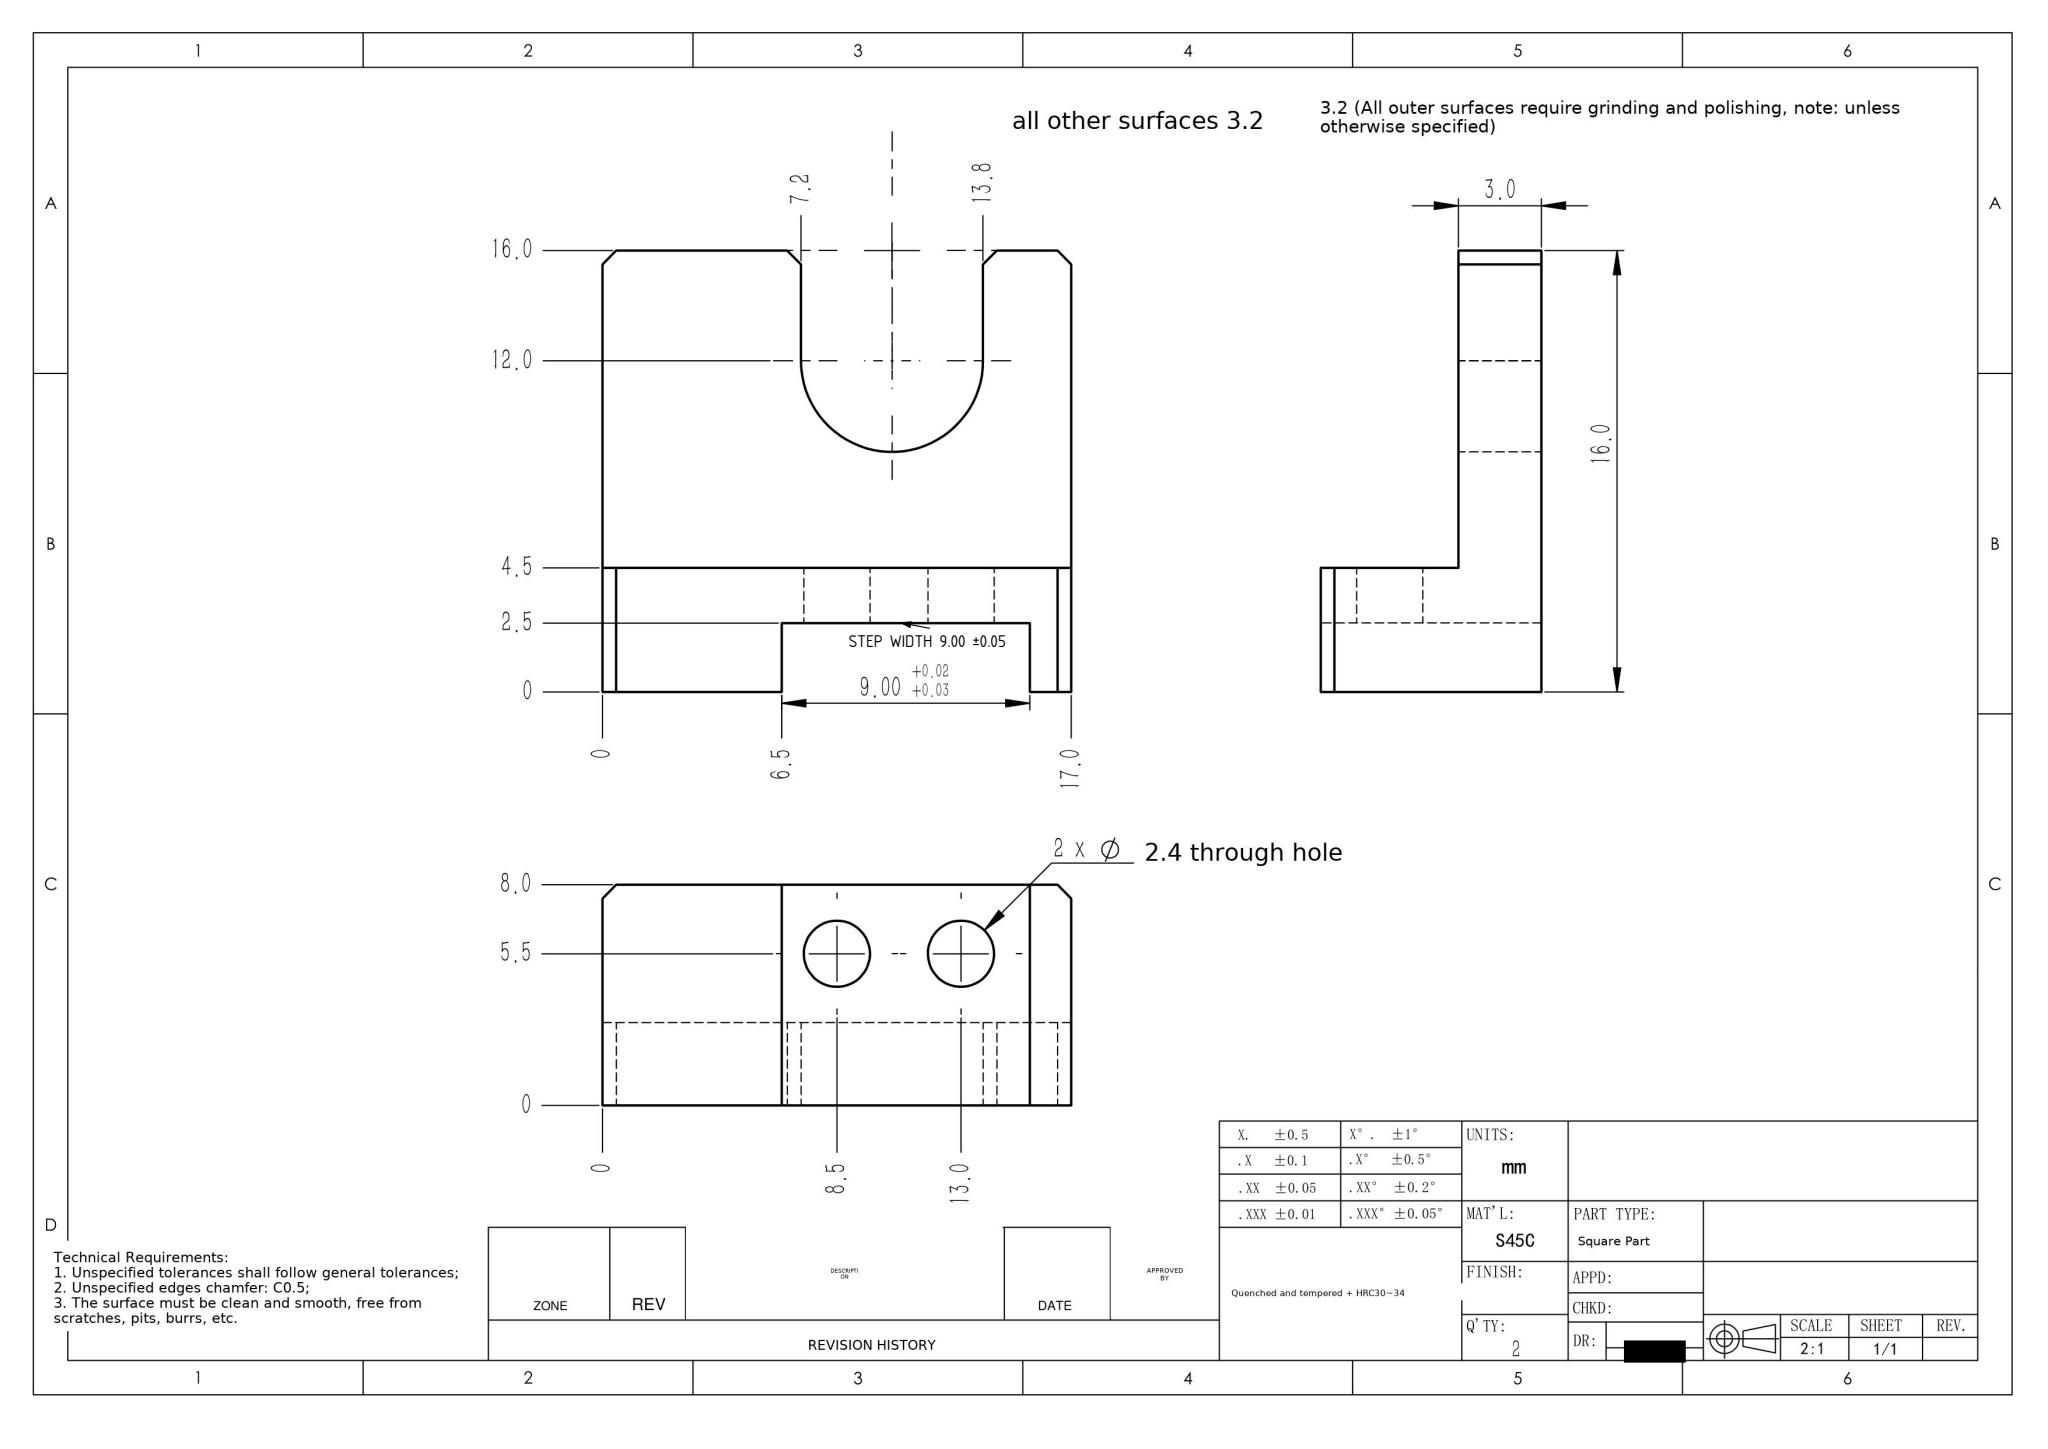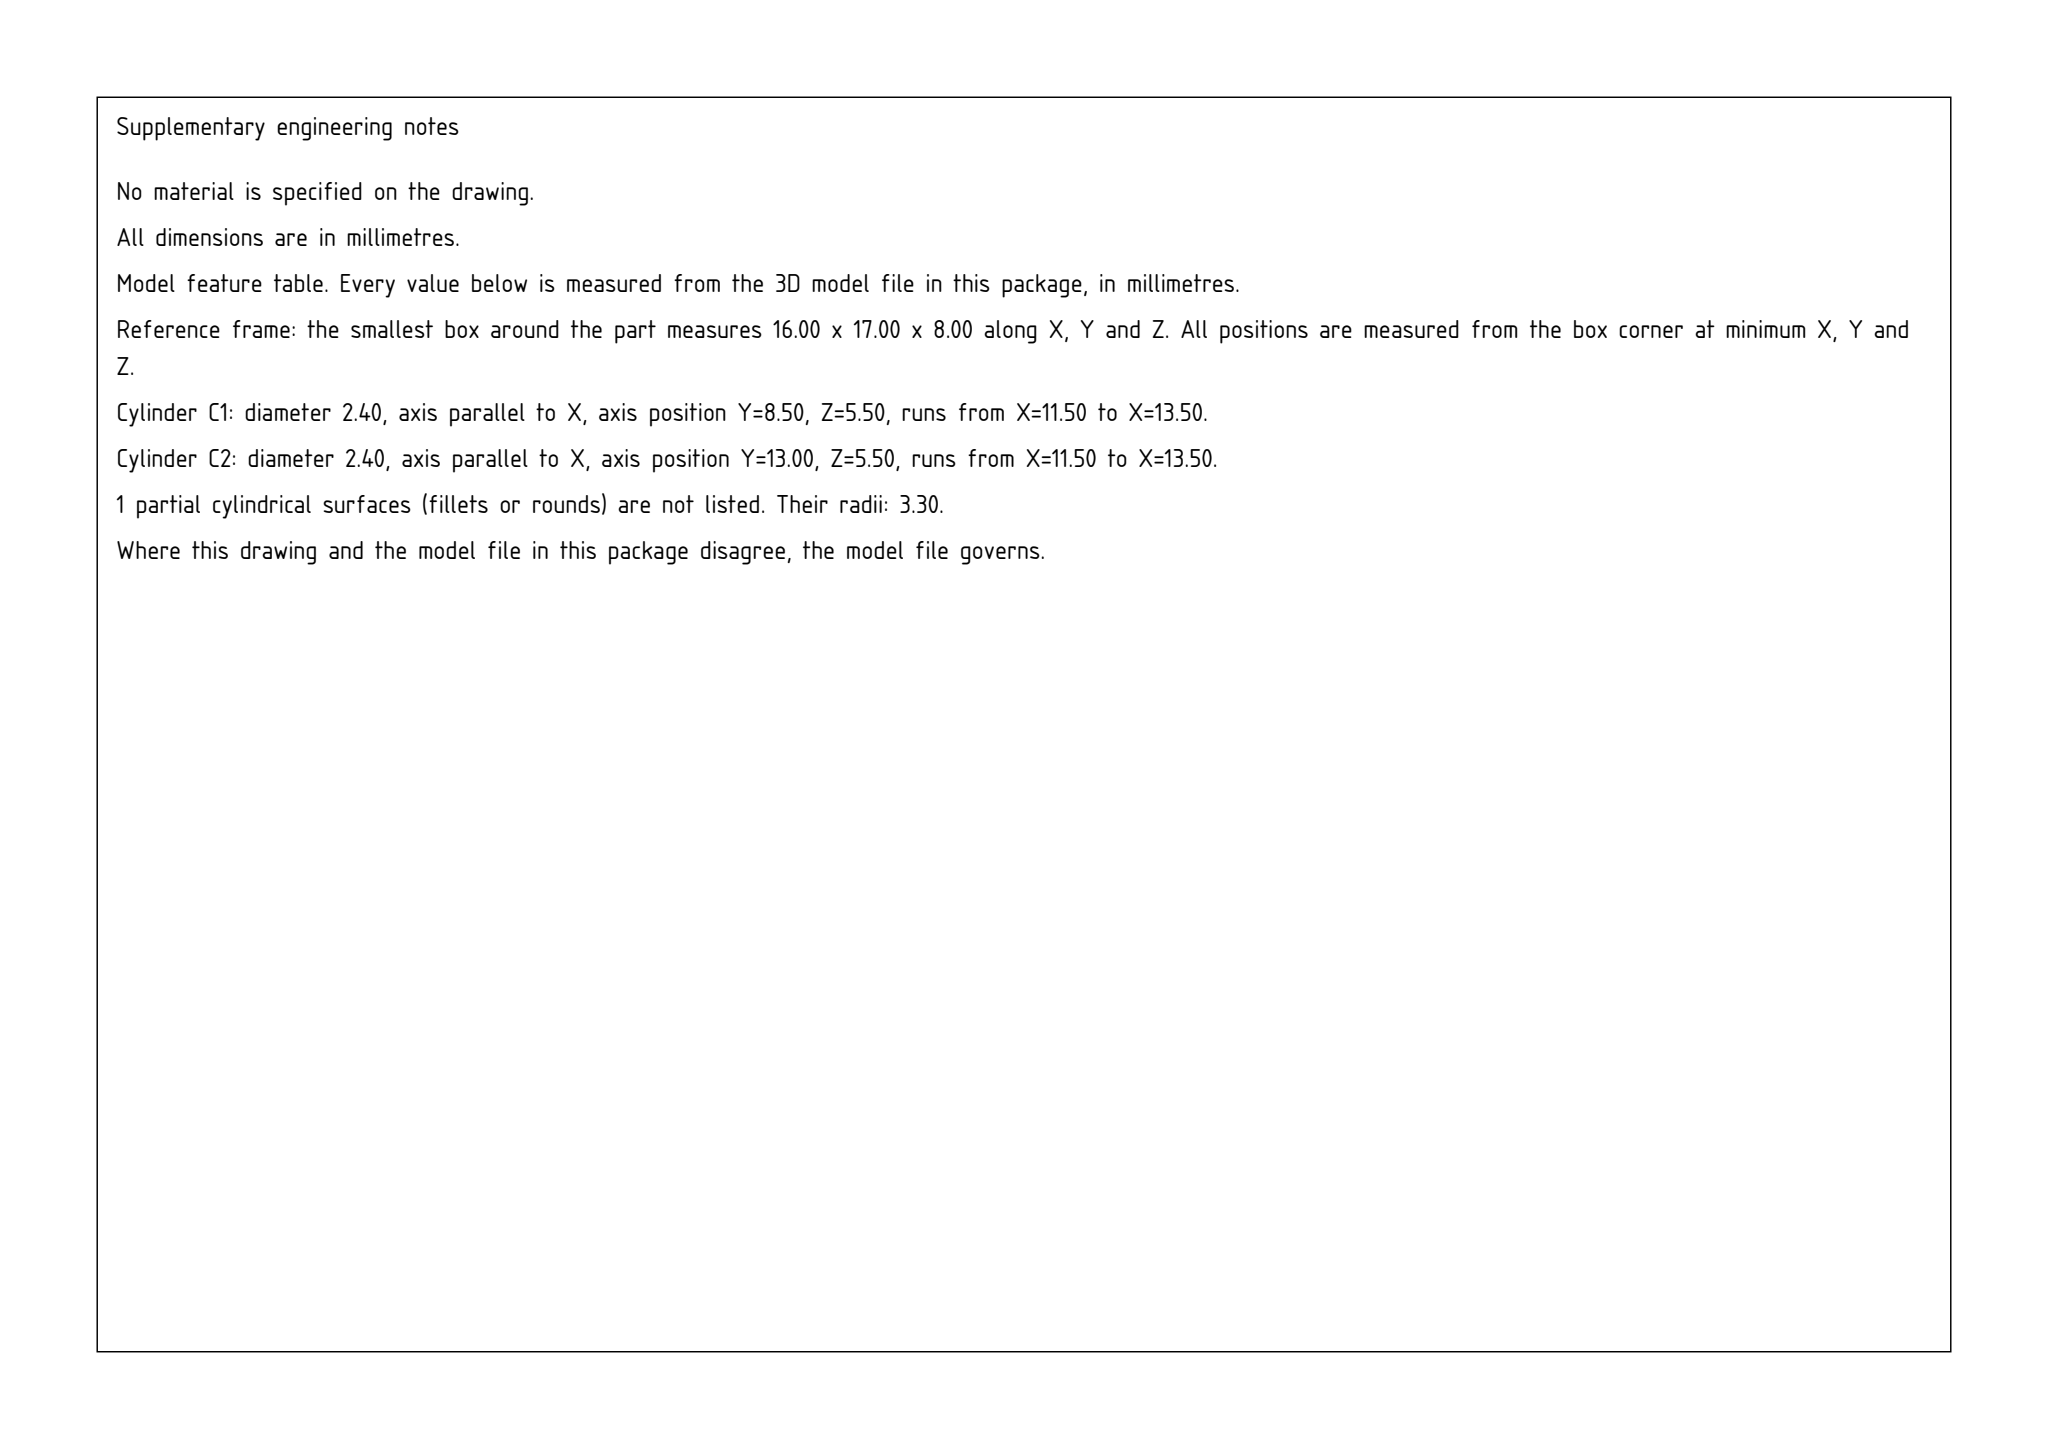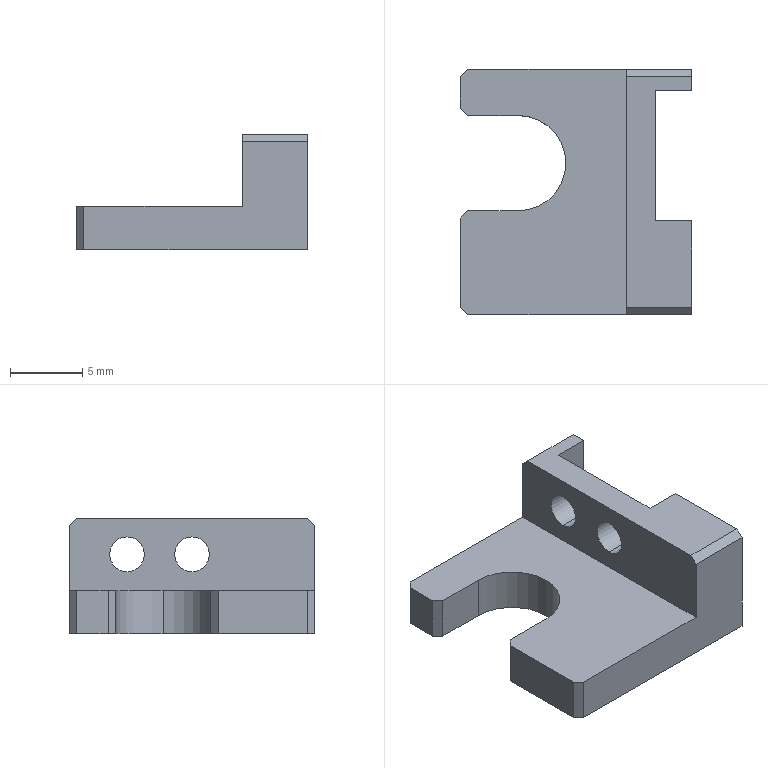Part | SolidWorks | mm | material S45C | 1 solid | 27 faces | box 16 x 17 x 8 mm | volume 867 mm3 | plane 21 | cylinder 6 | commonest cylinder face diameters 2.4 x4 6.6 x2
Drawing notes:
FRONT VIEW: STEP WIDTH 9.00 (FROM 6.5 TO 15.5), TOL ±0.05 | from the solid: Planes y=6.5 and y=15.5 (x 13.5-16.0, z 0-8) give step width 15.5-6.5=9.00; .XX tol block ±0.05
build123d program:
from build123d import *

# Parameters (mm, degrees)
SKETCH1_W            = 16
SKETCH1_H            = 17
BOSS_EXTRUDE1_DEPTH  = 8
SKETCH2_W            = 11.5
SKETCH2_H            = 17
CUT_EXTRUDE1_DEPTH   = 5
CUT_EXTRUDE2_DEPTH   = 19.795
SKETCH5_W            = 8
SKETCH5_H            = 9
CUT_EXTRUDE3_DEPTH   = 2.5
M2_CLEARANCE_HOLE1_D = 2.4
CHAMFER1_SIZE        = 0.5


with BuildPart() as part:
    # Sketch1 → Boss-Extrude1 (new body)
    with BuildSketch(Plane.XY):
        with Locations((-8, 0)):
            Rectangle(SKETCH1_W, SKETCH1_H)
    extrude(amount=BOSS_EXTRUDE1_DEPTH)

    # Sketch2 → Cut-Extrude1 (cut)
    with BuildSketch(Plane.XY.offset(8)):
        with Locations((-10.25, 0)):
            Rectangle(SKETCH2_W, SKETCH2_H)
    extrude(amount=-CUT_EXTRUDE1_DEPTH, mode=Mode.SUBTRACT)

    # Sketch3 → Cut-Extrude2 (cut, through all)
    with BuildSketch(Plane.XY.offset(3)):
        with BuildLine():
            Line((-16, 5.3), (-12, 5.3))
            ThreePointArc((-12, 5.3), (-8.7, 2), (-12, -1.3))
            Line((-12, -1.3), (-16, -1.3))
            ThreePointArc((-16, -1.3), (-19.3, 2), (-16, 5.3))
        make_face()
    extrude(amount=-CUT_EXTRUDE2_DEPTH, mode=Mode.SUBTRACT)

    # Sketch5 → Cut-Extrude3 (cut)
    with BuildSketch(Plane(origin=(0, 0, 0), x_dir=(0, 0, -1), z_dir=(1, 0, 0))):
        with Locations((-4, 2.5)):
            Rectangle(SKETCH5_W, SKETCH5_H)
    extrude(amount=-CUT_EXTRUDE3_DEPTH, mode=Mode.SUBTRACT)

    # M2 Clearance Hole1 (through all)
    with Locations(Plane.ZY.offset(4.5)):
        with Locations((5.5, 4.5), (5.5, 0)):
            Hole(M2_CLEARANCE_HOLE1_D / 2)

    # Chamfer1
    chamfer1_edges = [part.edges().sort_by_distance(p)[0] for p in [
        (-2.25, -8.5, 8),
        (-16, -8.5, 1.5),
        (-16, 8.5, 1.5),
        (-16, -1.3, 1.5),
        (-16, 5.3, 1.5),
        (-2.25, 8.5, 8),
    ]]
    chamfer(chamfer1_edges, length=CHAMFER1_SIZE)


solid = part.part
STEP:
#1=CARTESIAN_POINT('',(-2.5,4.5,4.3));
#2=VERTEX_POINT('',#1);
#3=CARTESIAN_POINT('',(-2.5,4.5,6.7));
#4=VERTEX_POINT('',#3);
#5=CARTESIAN_POINT('',(-2.5,4.5,5.5));
#6=DIRECTION('',(-1.,0.,0.));
#7=DIRECTION('',(0.,0.,1.));
#8=AXIS2_PLACEMENT_3D('',#5,#6,#7);
#9=CIRCLE('',#8,1.2);
#10=EDGE_CURVE('',#2,#4,#9,.T.);
#11=ORIENTED_EDGE('',*,*,#10,.F.);
#12=CARTESIAN_POINT('',(-4.5,4.5,4.3));
#13=VERTEX_POINT('',#12);
#14=CARTESIAN_POINT('',(-4.5,4.5,4.3));
#15=DIRECTION('',(-1.,0.,0.));
#16=VECTOR('',#15,1000.);
#17=LINE('',#14,#16);
#18=EDGE_CURVE('',#2,#13,#17,.T.);
#19=ORIENTED_EDGE('',*,*,#18,.T.);
#20=CARTESIAN_POINT('',(-4.5,4.5,6.7));
#21=VERTEX_POINT('',#20);
#22=CARTESIAN_POINT('',(-4.5,4.5,5.5));
#23=DIRECTION('',(-1.,0.,0.));
#24=DIRECTION('',(0.,0.,1.));
#25=AXIS2_PLACEMENT_3D('',#22,#23,#24);
#26=CIRCLE('',#25,1.2);
#27=EDGE_CURVE('',#13,#21,#26,.T.);
#28=ORIENTED_EDGE('',*,*,#27,.T.);
#29=CARTESIAN_POINT('',(-4.5,4.5,6.7));
#30=DIRECTION('',(-1.,0.,0.));
#31=VECTOR('',#30,1000.);
#32=LINE('',#29,#31);
#33=EDGE_CURVE('',#4,#21,#32,.T.);
#34=ORIENTED_EDGE('',*,*,#33,.F.);
#35=EDGE_LOOP('',(#11,#19,#28,#34));
#36=FACE_OUTER_BOUND('',#35,.T.);
#37=CARTESIAN_POINT('',(-4.5,4.5,5.5));
#38=DIRECTION('',(-1.,0.,0.));
#39=DIRECTION('',(0.,0.,1.));
#40=AXIS2_PLACEMENT_3D('',#37,#38,#39);
#41=CYLINDRICAL_SURFACE('',#40,1.2);
#42=ADVANCED_FACE('',(#36),#41,.F.);
#43=CARTESIAN_POINT('',(-2.5,0.,4.3));
#44=VERTEX_POINT('',#43);
#45=CARTESIAN_POINT('',(-2.5,0.,6.7));
#46=VERTEX_POINT('',#45);
#47=CARTESIAN_POINT('',(-2.5,0.,5.5));
#48=DIRECTION('',(-1.,0.,0.));
#49=DIRECTION('',(0.,0.,1.));
#50=AXIS2_PLACEMENT_3D('',#47,#48,#49);
#51=CIRCLE('',#50,1.2);
#52=EDGE_CURVE('',#44,#46,#51,.T.);
#53=ORIENTED_EDGE('',*,*,#52,.F.);
#54=CARTESIAN_POINT('',(-4.5,0.,4.3));
#55=VERTEX_POINT('',#54);
#56=CARTESIAN_POINT('',(-4.5,0.,4.3));
#57=DIRECTION('',(-1.,0.,0.));
#58=VECTOR('',#57,1000.);
#59=LINE('',#56,#58);
#60=EDGE_CURVE('',#44,#55,#59,.T.);
#61=ORIENTED_EDGE('',*,*,#60,.T.);
#62=CARTESIAN_POINT('',(-4.5,0.,6.7));
#63=VERTEX_POINT('',#62);
#64=CARTESIAN_POINT('',(-4.5,0.,5.5));
#65=DIRECTION('',(-1.,0.,0.));
#66=DIRECTION('',(0.,0.,1.));
#67=AXIS2_PLACEMENT_3D('',#64,#65,#66);
#68=CIRCLE('',#67,1.2);
#69=EDGE_CURVE('',#55,#63,#68,.T.);
#70=ORIENTED_EDGE('',*,*,#69,.T.);
#71=CARTESIAN_POINT('',(-4.5,0.,6.7));
#72=DIRECTION('',(-1.,0.,0.));
#73=VECTOR('',#72,1000.);
#74=LINE('',#71,#73);
#75=EDGE_CURVE('',#46,#63,#74,.T.);
#76=ORIENTED_EDGE('',*,*,#75,.F.);
#77=EDGE_LOOP('',(#53,#61,#70,#76));
#78=FACE_OUTER_BOUND('',#77,.T.);
#79=CARTESIAN_POINT('',(-4.5,0.,5.5));
#80=DIRECTION('',(-1.,0.,0.));
#81=DIRECTION('',(0.,0.,1.));
#82=AXIS2_PLACEMENT_3D('',#79,#80,#81);
#83=CYLINDRICAL_SURFACE('',#82,1.2);
#84=ADVANCED_FACE('',(#78),#83,.F.);
#85=CARTESIAN_POINT('',(-8.7,2.,0.));
#86=VERTEX_POINT('',#85);
#87=CARTESIAN_POINT('',(-12.,5.3,0.));
#88=VERTEX_POINT('',#87);
#89=CARTESIAN_POINT('',(-12.,2.,0.));
#90=DIRECTION('',(0.,0.,1.));
#91=DIRECTION('',(1.,0.,0.));
#92=AXIS2_PLACEMENT_3D('',#89,#90,#91);
#93=CIRCLE('',#92,3.3);
#94=EDGE_CURVE('',#86,#88,#93,.T.);
#95=ORIENTED_EDGE('',*,*,#94,.F.);
#96=CARTESIAN_POINT('',(-8.7,2.,3.));
#97=VERTEX_POINT('',#96);
#98=CARTESIAN_POINT('',(-8.7,2.,0.));
#99=DIRECTION('',(0.,0.,1.));
#100=VECTOR('',#99,1000.);
#101=LINE('',#98,#100);
#102=EDGE_CURVE('',#86,#97,#101,.T.);
#103=ORIENTED_EDGE('',*,*,#102,.T.);
#104=CARTESIAN_POINT('',(-12.,5.3,3.));
#105=VERTEX_POINT('',#104);
#106=CARTESIAN_POINT('',(-12.,2.,3.));
#107=DIRECTION('',(0.,0.,1.));
#108=DIRECTION('',(1.,0.,0.));
#109=AXIS2_PLACEMENT_3D('',#106,#107,#108);
#110=CIRCLE('',#109,3.3);
#111=EDGE_CURVE('',#97,#105,#110,.T.);
#112=ORIENTED_EDGE('',*,*,#111,.T.);
#113=CARTESIAN_POINT('',(-12.,5.3,0.));
#114=DIRECTION('',(0.,0.,1.));
#115=VECTOR('',#114,1000.);
#116=LINE('',#113,#115);
#117=EDGE_CURVE('',#88,#105,#116,.T.);
#118=ORIENTED_EDGE('',*,*,#117,.F.);
#119=EDGE_LOOP('',(#95,#103,#112,#118));
#120=FACE_OUTER_BOUND('',#119,.T.);
#121=CARTESIAN_POINT('',(-12.,2.,0.));
#122=DIRECTION('',(0.,0.,1.));
#123=DIRECTION('',(1.,0.,0.));
#124=AXIS2_PLACEMENT_3D('',#121,#122,#123);
#125=CYLINDRICAL_SURFACE('',#124,3.3);
#126=ADVANCED_FACE('',(#120),#125,.F.);
#127=CARTESIAN_POINT('',(0.,-8.,8.));
#128=VERTEX_POINT('',#127);
#129=CARTESIAN_POINT('',(0.,-2.,8.));
#130=VERTEX_POINT('',#129);
#131=CARTESIAN_POINT('',(0.,8.5,8.));
#132=DIRECTION('',(0.,1.,0.));
#133=VECTOR('',#132,1000.);
#134=LINE('',#131,#133);
#135=EDGE_CURVE('',#128,#130,#134,.T.);
#136=ORIENTED_EDGE('',*,*,#135,.F.);
#137=CARTESIAN_POINT('',(0.,-8.5,7.5));
#138=VERTEX_POINT('',#137);
#139=CARTESIAN_POINT('',(0.,-8.,8.));
#140=DIRECTION('',(0.,-0.7071,-0.7071));
#141=VECTOR('',#140,1000.);
#142=LINE('',#139,#141);
#143=EDGE_CURVE('',#128,#138,#142,.T.);
#144=ORIENTED_EDGE('',*,*,#143,.T.);
#145=CARTESIAN_POINT('',(0.,-8.5,0.));
#146=VERTEX_POINT('',#145);
#147=CARTESIAN_POINT('',(0.,-8.5,8.));
#148=DIRECTION('',(0.,0.,-1.));
#149=VECTOR('',#148,1000.);
#150=LINE('',#147,#149);
#151=EDGE_CURVE('',#138,#146,#150,.T.);
#152=ORIENTED_EDGE('',*,*,#151,.T.);
#153=CARTESIAN_POINT('',(0.,-2.,-0.));
#154=VERTEX_POINT('',#153);
#155=CARTESIAN_POINT('',(0.,8.5,0.));
#156=DIRECTION('',(0.,1.,0.));
#157=VECTOR('',#156,1000.);
#158=LINE('',#155,#157);
#159=EDGE_CURVE('',#146,#154,#158,.T.);
#160=ORIENTED_EDGE('',*,*,#159,.T.);
#161=CARTESIAN_POINT('',(0.,-2.,-0.));
#162=DIRECTION('',(0.,0.,-1.));
#163=VECTOR('',#162,1000.);
#164=LINE('',#161,#163);
#165=EDGE_CURVE('',#130,#154,#164,.T.);
#166=ORIENTED_EDGE('',*,*,#165,.F.);
#167=EDGE_LOOP('',(#136,#144,#152,#160,#166));
#168=FACE_OUTER_BOUND('',#167,.T.);
#169=CARTESIAN_POINT('',(0.,8.5,8.));
#170=DIRECTION('',(-1.,0.,0.));
#171=DIRECTION('',(0.,0.,1.));
#172=AXIS2_PLACEMENT_3D('',#169,#170,#171);
#173=PLANE('',#172);
#174=ADVANCED_FACE('',(#168),#173,.F.);
#175=CARTESIAN_POINT('',(-16.,8.,0.));
#176=VERTEX_POINT('',#175);
#177=CARTESIAN_POINT('',(-16.,5.8,0.));
#178=VERTEX_POINT('',#177);
#179=CARTESIAN_POINT('',(-16.,8.5,0.));
#180=DIRECTION('',(0.,-1.,0.));
#181=VECTOR('',#180,1000.);
#182=LINE('',#179,#181);
#183=EDGE_CURVE('',#176,#178,#182,.T.);
#184=ORIENTED_EDGE('',*,*,#183,.T.);
#185=CARTESIAN_POINT('',(-16.,5.8,3.));
#186=VERTEX_POINT('',#185);
#187=CARTESIAN_POINT('',(-16.,5.8,8.));
#188=DIRECTION('',(0.,0.,1.));
#189=VECTOR('',#188,1000.);
#190=LINE('',#187,#189);
#191=EDGE_CURVE('',#178,#186,#190,.T.);
#192=ORIENTED_EDGE('',*,*,#191,.T.);
#193=CARTESIAN_POINT('',(-16.,8.,3.));
#194=VERTEX_POINT('',#193);
#195=CARTESIAN_POINT('',(-16.,8.5,3.));
#196=DIRECTION('',(0.,-1.,0.));
#197=VECTOR('',#196,1000.);
#198=LINE('',#195,#197);
#199=EDGE_CURVE('',#194,#186,#198,.T.);
#200=ORIENTED_EDGE('',*,*,#199,.F.);
#201=CARTESIAN_POINT('',(-16.,8.,8.));
#202=DIRECTION('',(0.,0.,-1.));
#203=VECTOR('',#202,1000.);
#204=LINE('',#201,#203);
#205=EDGE_CURVE('',#194,#176,#204,.T.);
#206=ORIENTED_EDGE('',*,*,#205,.T.);
#207=EDGE_LOOP('',(#184,#192,#200,#206));
#208=FACE_OUTER_BOUND('',#207,.T.);
#209=CARTESIAN_POINT('',(-16.,8.5,8.));
#210=DIRECTION('',(1.,0.,0.));
#211=DIRECTION('',(0.,0.,-1.));
#212=AXIS2_PLACEMENT_3D('',#209,#210,#211);
#213=PLANE('',#212);
#214=ADVANCED_FACE('',(#208),#213,.F.);
#215=CARTESIAN_POINT('',(0.,8.5,7.5));
#216=VERTEX_POINT('',#215);
#217=CARTESIAN_POINT('',(0.,8.5,0.));
#218=VERTEX_POINT('',#217);
#219=CARTESIAN_POINT('',(0.,8.5,8.));
#220=DIRECTION('',(0.,0.,-1.));
#221=VECTOR('',#220,1000.);
#222=LINE('',#219,#221);
#223=EDGE_CURVE('',#216,#218,#222,.T.);
#224=ORIENTED_EDGE('',*,*,#223,.F.);
#225=CARTESIAN_POINT('',(0.,8.,8.));
#226=VERTEX_POINT('',#225);
#227=CARTESIAN_POINT('',(0.,8.,8.));
#228=DIRECTION('',(0.,-0.7071,0.7071));
#229=VECTOR('',#228,1000.);
#230=LINE('',#227,#229);
#231=EDGE_CURVE('',#216,#226,#230,.T.);
#232=ORIENTED_EDGE('',*,*,#231,.T.);
#233=CARTESIAN_POINT('',(0.,7.,8.));
#234=VERTEX_POINT('',#233);
#235=CARTESIAN_POINT('',(0.,8.5,8.));
#236=DIRECTION('',(0.,1.,0.));
#237=VECTOR('',#236,1000.);
#238=LINE('',#235,#237);
#239=EDGE_CURVE('',#234,#226,#238,.T.);
#240=ORIENTED_EDGE('',*,*,#239,.F.);
#241=CARTESIAN_POINT('',(0.,7.,0.));
#242=VERTEX_POINT('',#241);
#243=CARTESIAN_POINT('',(0.,7.,0.));
#244=DIRECTION('',(0.,-0.,1.));
#245=VECTOR('',#244,1000.);
#246=LINE('',#243,#245);
#247=EDGE_CURVE('',#242,#234,#246,.T.);
#248=ORIENTED_EDGE('',*,*,#247,.F.);
#249=CARTESIAN_POINT('',(0.,8.5,0.));
#250=DIRECTION('',(0.,1.,0.));
#251=VECTOR('',#250,1000.);
#252=LINE('',#249,#251);
#253=EDGE_CURVE('',#242,#218,#252,.T.);
#254=ORIENTED_EDGE('',*,*,#253,.T.);
#255=EDGE_LOOP('',(#224,#232,#240,#248,#254));
#256=FACE_OUTER_BOUND('',#255,.T.);
#257=CARTESIAN_POINT('',(0.,8.5,8.));
#258=DIRECTION('',(-1.,0.,0.));
#259=DIRECTION('',(0.,0.,1.));
#260=AXIS2_PLACEMENT_3D('',#257,#258,#259);
#261=PLANE('',#260);
#262=ADVANCED_FACE('',(#256),#261,.F.);
#263=CARTESIAN_POINT('',(-4.5,8.5,3.));
#264=VERTEX_POINT('',#263);
#265=CARTESIAN_POINT('',(-4.5,8.5,7.5));
#266=VERTEX_POINT('',#265);
#267=CARTESIAN_POINT('',(-4.5,8.5,-20.524));
#268=DIRECTION('',(0.,0.,1.));
#269=VECTOR('',#268,1000.);
#270=LINE('',#267,#269);
#271=EDGE_CURVE('',#264,#266,#270,.T.);
#272=ORIENTED_EDGE('',*,*,#271,.T.);
#273=CARTESIAN_POINT('',(0.,8.5,7.5));
#274=DIRECTION('',(1.,0.,0.));
#275=VECTOR('',#274,1000.);
#276=LINE('',#273,#275);
#277=EDGE_CURVE('',#266,#216,#276,.T.);
#278=ORIENTED_EDGE('',*,*,#277,.T.);
#279=ORIENTED_EDGE('',*,*,#223,.T.);
#280=CARTESIAN_POINT('',(-15.5,8.5,0.));
#281=VERTEX_POINT('',#280);
#282=CARTESIAN_POINT('',(0.,8.5,0.));
#283=DIRECTION('',(-1.,-0.,0.));
#284=VECTOR('',#283,1000.);
#285=LINE('',#282,#284);
#286=EDGE_CURVE('',#218,#281,#285,.T.);
#287=ORIENTED_EDGE('',*,*,#286,.T.);
#288=CARTESIAN_POINT('',(-15.5,8.5,3.));
#289=VERTEX_POINT('',#288);
#290=CARTESIAN_POINT('',(-15.5,8.5,8.));
#291=DIRECTION('',(0.,0.,1.));
#292=VECTOR('',#291,1000.);
#293=LINE('',#290,#292);
#294=EDGE_CURVE('',#281,#289,#293,.T.);
#295=ORIENTED_EDGE('',*,*,#294,.T.);
#296=CARTESIAN_POINT('',(-16.,8.5,3.));
#297=DIRECTION('',(-1.,0.,0.));
#298=VECTOR('',#297,1000.);
#299=LINE('',#296,#298);
#300=EDGE_CURVE('',#264,#289,#299,.T.);
#301=ORIENTED_EDGE('',*,*,#300,.F.);
#302=EDGE_LOOP('',(#272,#278,#279,#287,#295,#301));
#303=FACE_OUTER_BOUND('',#302,.T.);
#304=CARTESIAN_POINT('',(0.,8.5,8.));
#305=DIRECTION('',(0.,-1.,0.));
#306=DIRECTION('',(1.,0.,0.));
#307=AXIS2_PLACEMENT_3D('',#304,#305,#306);
#308=PLANE('',#307);
#309=ADVANCED_FACE('',(#303),#308,.F.);
#310=CARTESIAN_POINT('',(-16.,-1.8,3.));
#311=VERTEX_POINT('',#310);
#312=CARTESIAN_POINT('',(-16.,-8.,3.));
#313=VERTEX_POINT('',#312);
#314=CARTESIAN_POINT('',(-16.,8.5,3.));
#315=DIRECTION('',(0.,-1.,0.));
#316=VECTOR('',#315,1000.);
#317=LINE('',#314,#316);
#318=EDGE_CURVE('',#311,#313,#317,.T.);
#319=ORIENTED_EDGE('',*,*,#318,.F.);
#320=CARTESIAN_POINT('',(-16.,-1.8,0.));
#321=VERTEX_POINT('',#320);
#322=CARTESIAN_POINT('',(-16.,-1.8,8.));
#323=DIRECTION('',(0.,0.,-1.));
#324=VECTOR('',#323,1000.);
#325=LINE('',#322,#324);
#326=EDGE_CURVE('',#311,#321,#325,.T.);
#327=ORIENTED_EDGE('',*,*,#326,.T.);
#328=CARTESIAN_POINT('',(-16.,-8.,0.));
#329=VERTEX_POINT('',#328);
#330=CARTESIAN_POINT('',(-16.,8.5,0.));
#331=DIRECTION('',(0.,-1.,0.));
#332=VECTOR('',#331,1000.);
#333=LINE('',#330,#332);
#334=EDGE_CURVE('',#321,#329,#333,.T.);
#335=ORIENTED_EDGE('',*,*,#334,.T.);
#336=CARTESIAN_POINT('',(-16.,-8.,8.));
#337=DIRECTION('',(0.,0.,1.));
#338=VECTOR('',#337,1000.);
#339=LINE('',#336,#338);
#340=EDGE_CURVE('',#329,#313,#339,.T.);
#341=ORIENTED_EDGE('',*,*,#340,.T.);
#342=EDGE_LOOP('',(#319,#327,#335,#341));
#343=FACE_OUTER_BOUND('',#342,.T.);
#344=CARTESIAN_POINT('',(-16.,8.5,8.));
#345=DIRECTION('',(1.,0.,0.));
#346=DIRECTION('',(0.,0.,-1.));
#347=AXIS2_PLACEMENT_3D('',#344,#345,#346);
#348=PLANE('',#347);
#349=ADVANCED_FACE('',(#343),#348,.F.);
#350=ORIENTED_EDGE('',*,*,#151,.F.);
#351=CARTESIAN_POINT('',(-4.5,-8.5,7.5));
#352=VERTEX_POINT('',#351);
#353=CARTESIAN_POINT('',(0.,-8.5,7.5));
#354=DIRECTION('',(-1.,0.,0.));
#355=VECTOR('',#354,1000.);
#356=LINE('',#353,#355);
#357=EDGE_CURVE('',#138,#352,#356,.T.);
#358=ORIENTED_EDGE('',*,*,#357,.T.);
#359=CARTESIAN_POINT('',(-4.5,-8.5,3.));
#360=VERTEX_POINT('',#359);
#361=CARTESIAN_POINT('',(-4.5,-8.5,-20.524));
#362=DIRECTION('',(0.,0.,1.));
#363=VECTOR('',#362,1000.);
#364=LINE('',#361,#363);
#365=EDGE_CURVE('',#360,#352,#364,.T.);
#366=ORIENTED_EDGE('',*,*,#365,.F.);
#367=CARTESIAN_POINT('',(-15.5,-8.5,3.));
#368=VERTEX_POINT('',#367);
#369=CARTESIAN_POINT('',(-16.,-8.5,3.));
#370=DIRECTION('',(1.,0.,0.));
#371=VECTOR('',#370,1000.);
#372=LINE('',#369,#371);
#373=EDGE_CURVE('',#368,#360,#372,.T.);
#374=ORIENTED_EDGE('',*,*,#373,.F.);
#375=CARTESIAN_POINT('',(-15.5,-8.5,0.));
#376=VERTEX_POINT('',#375);
#377=CARTESIAN_POINT('',(-15.5,-8.5,8.));
#378=DIRECTION('',(0.,0.,-1.));
#379=VECTOR('',#378,1000.);
#380=LINE('',#377,#379);
#381=EDGE_CURVE('',#368,#376,#380,.T.);
#382=ORIENTED_EDGE('',*,*,#381,.T.);
#383=CARTESIAN_POINT('',(0.,-8.5,0.));
#384=DIRECTION('',(1.,-0.,0.));
#385=VECTOR('',#384,1000.);
#386=LINE('',#383,#385);
#387=EDGE_CURVE('',#376,#146,#386,.T.);
#388=ORIENTED_EDGE('',*,*,#387,.T.);
#389=EDGE_LOOP('',(#350,#358,#366,#374,#382,#388));
#390=FACE_OUTER_BOUND('',#389,.T.);
#391=CARTESIAN_POINT('',(0.,-8.5,8.));
#392=DIRECTION('',(0.,1.,0.));
#393=DIRECTION('',(-1.,0.,0.));
#394=AXIS2_PLACEMENT_3D('',#391,#392,#393);
#395=PLANE('',#394);
#396=ADVANCED_FACE('',(#390),#395,.F.);
#397=CARTESIAN_POINT('',(-4.5,-8.,8.));
#398=VERTEX_POINT('',#397);
#399=CARTESIAN_POINT('',(-4.5,8.,8.));
#400=VERTEX_POINT('',#399);
#401=CARTESIAN_POINT('',(-4.5,8.5,8.));
#402=DIRECTION('',(-0.,1.,0.));
#403=VECTOR('',#402,1000.);
#404=LINE('',#401,#403);
#405=EDGE_CURVE('',#398,#400,#404,.T.);
#406=ORIENTED_EDGE('',*,*,#405,.F.);
#407=CARTESIAN_POINT('',(-0.,-8.,8.));
#408=DIRECTION('',(1.,-0.,0.));
#409=VECTOR('',#408,1000.);
#410=LINE('',#407,#409);
#411=EDGE_CURVE('',#398,#128,#410,.T.);
#412=ORIENTED_EDGE('',*,*,#411,.T.);
#413=ORIENTED_EDGE('',*,*,#135,.T.);
#414=CARTESIAN_POINT('',(-2.5,-2.,8.));
#415=VERTEX_POINT('',#414);
#416=CARTESIAN_POINT('',(-2.5,-2.,8.));
#417=DIRECTION('',(1.,0.,0.));
#418=VECTOR('',#417,1000.);
#419=LINE('',#416,#418);
#420=EDGE_CURVE('',#415,#130,#419,.T.);
#421=ORIENTED_EDGE('',*,*,#420,.F.);
#422=CARTESIAN_POINT('',(-2.5,7.,8.));
#423=VERTEX_POINT('',#422);
#424=CARTESIAN_POINT('',(-2.5,7.,8.));
#425=DIRECTION('',(0.,-1.,0.));
#426=VECTOR('',#425,1000.);
#427=LINE('',#424,#426);
#428=EDGE_CURVE('',#423,#415,#427,.T.);
#429=ORIENTED_EDGE('',*,*,#428,.F.);
#430=CARTESIAN_POINT('',(-2.5,7.,8.));
#431=DIRECTION('',(1.,0.,0.));
#432=VECTOR('',#431,1000.);
#433=LINE('',#430,#432);
#434=EDGE_CURVE('',#423,#234,#433,.T.);
#435=ORIENTED_EDGE('',*,*,#434,.T.);
#436=ORIENTED_EDGE('',*,*,#239,.T.);
#437=CARTESIAN_POINT('',(-0.,8.,8.));
#438=DIRECTION('',(-1.,-0.,0.));
#439=VECTOR('',#438,1000.);
#440=LINE('',#437,#439);
#441=EDGE_CURVE('',#226,#400,#440,.T.);
#442=ORIENTED_EDGE('',*,*,#441,.T.);
#443=EDGE_LOOP('',(#406,#412,#413,#421,#429,#435,#436,#442));
#444=FACE_OUTER_BOUND('',#443,.T.);
#445=CARTESIAN_POINT('',(0.,0.,8.));
#446=DIRECTION('',(0.,0.,-1.));
#447=DIRECTION('',(-1.,0.,0.));
#448=AXIS2_PLACEMENT_3D('',#445,#446,#447);
#449=PLANE('',#448);
#450=ADVANCED_FACE('',(#444),#449,.F.);
#451=CARTESIAN_POINT('',(-15.5,5.3,0.));
#452=VERTEX_POINT('',#451);
#453=CARTESIAN_POINT('',(-16.,5.3,0.));
#454=DIRECTION('',(-1.,0.,0.));
#455=VECTOR('',#454,1000.);
#456=LINE('',#453,#455);
#457=EDGE_CURVE('',#88,#452,#456,.T.);
#458=ORIENTED_EDGE('',*,*,#457,.T.);
#459=CARTESIAN_POINT('',(-5.1,-5.1,0.));
#460=DIRECTION('',(-0.7071,0.7071,0.));
#461=VECTOR('',#460,1000.);
#462=LINE('',#459,#461);
#463=EDGE_CURVE('',#452,#178,#462,.T.);
#464=ORIENTED_EDGE('',*,*,#463,.T.);
#465=ORIENTED_EDGE('',*,*,#183,.F.);
#466=CARTESIAN_POINT('',(-12.,12.,0.));
#467=DIRECTION('',(0.7071,0.7071,0.));
#468=VECTOR('',#467,1000.);
#469=LINE('',#466,#468);
#470=EDGE_CURVE('',#176,#281,#469,.T.);
#471=ORIENTED_EDGE('',*,*,#470,.T.);
#472=ORIENTED_EDGE('',*,*,#286,.F.);
#473=ORIENTED_EDGE('',*,*,#253,.F.);
#474=CARTESIAN_POINT('',(-2.5,7.,0.));
#475=VERTEX_POINT('',#474);
#476=CARTESIAN_POINT('',(-2.5,7.,0.));
#477=DIRECTION('',(1.,0.,0.));
#478=VECTOR('',#477,1000.);
#479=LINE('',#476,#478);
#480=EDGE_CURVE('',#475,#242,#479,.T.);
#481=ORIENTED_EDGE('',*,*,#480,.F.);
#482=CARTESIAN_POINT('',(-2.5,-2.,0.));
#483=VERTEX_POINT('',#482);
#484=CARTESIAN_POINT('',(-2.5,7.,0.));
#485=DIRECTION('',(0.,1.,0.));
#486=VECTOR('',#485,1000.);
#487=LINE('',#484,#486);
#488=EDGE_CURVE('',#483,#475,#487,.T.);
#489=ORIENTED_EDGE('',*,*,#488,.F.);
#490=CARTESIAN_POINT('',(-2.5,-2.,-0.));
#491=DIRECTION('',(1.,0.,0.));
#492=VECTOR('',#491,1000.);
#493=LINE('',#490,#492);
#494=EDGE_CURVE('',#483,#154,#493,.T.);
#495=ORIENTED_EDGE('',*,*,#494,.T.);
#496=ORIENTED_EDGE('',*,*,#159,.F.);
#497=ORIENTED_EDGE('',*,*,#387,.F.);
#498=CARTESIAN_POINT('',(-12.,-12.,0.));
#499=DIRECTION('',(-0.7071,0.7071,0.));
#500=VECTOR('',#499,1000.);
#501=LINE('',#498,#500);
#502=EDGE_CURVE('',#376,#329,#501,.T.);
#503=ORIENTED_EDGE('',*,*,#502,.T.);
#504=ORIENTED_EDGE('',*,*,#334,.F.);
#505=CARTESIAN_POINT('',(-15.5,-1.3,0.));
#506=VERTEX_POINT('',#505);
#507=CARTESIAN_POINT('',(-7.1,7.1,0.));
#508=DIRECTION('',(0.7071,0.7071,0.));
#509=VECTOR('',#508,1000.);
#510=LINE('',#507,#509);
#511=EDGE_CURVE('',#321,#506,#510,.T.);
#512=ORIENTED_EDGE('',*,*,#511,.T.);
#513=CARTESIAN_POINT('',(-12.,-1.3,0.));
#514=VERTEX_POINT('',#513);
#515=CARTESIAN_POINT('',(-16.,-1.3,0.));
#516=DIRECTION('',(1.,0.,0.));
#517=VECTOR('',#516,1000.);
#518=LINE('',#515,#517);
#519=EDGE_CURVE('',#506,#514,#518,.T.);
#520=ORIENTED_EDGE('',*,*,#519,.T.);
#521=CARTESIAN_POINT('',(-12.,2.,0.));
#522=DIRECTION('',(0.,0.,1.));
#523=DIRECTION('',(1.,0.,0.));
#524=AXIS2_PLACEMENT_3D('',#521,#522,#523);
#525=CIRCLE('',#524,3.3);
#526=EDGE_CURVE('',#514,#86,#525,.T.);
#527=ORIENTED_EDGE('',*,*,#526,.T.);
#528=ORIENTED_EDGE('',*,*,#94,.T.);
#529=EDGE_LOOP('',(#458,#464,#465,#471,#472,#473,#481,#489,#495,#496,#497,#503,#504,#512,#520,#527,#528));
#530=FACE_OUTER_BOUND('',#529,.T.);
#531=CARTESIAN_POINT('',(0.,0.,0.));
#532=DIRECTION('',(0.,0.,-1.));
#533=DIRECTION('',(-1.,0.,0.));
#534=AXIS2_PLACEMENT_3D('',#531,#532,#533);
#535=PLANE('',#534);
#536=ADVANCED_FACE('',(#530),#535,.T.);
#537=ORIENTED_EDGE('',*,*,#199,.T.);
#538=CARTESIAN_POINT('',(-15.5,5.3,3.));
#539=VERTEX_POINT('',#538);
#540=CARTESIAN_POINT('',(-16.,5.8,3.));
#541=DIRECTION('',(0.7071,-0.7071,0.));
#542=VECTOR('',#541,1000.);
#543=LINE('',#540,#542);
#544=EDGE_CURVE('',#186,#539,#543,.T.);
#545=ORIENTED_EDGE('',*,*,#544,.T.);
#546=CARTESIAN_POINT('',(-16.,5.3,3.));
#547=DIRECTION('',(-1.,0.,0.));
#548=VECTOR('',#547,1000.);
#549=LINE('',#546,#548);
#550=EDGE_CURVE('',#105,#539,#549,.T.);
#551=ORIENTED_EDGE('',*,*,#550,.F.);
#552=ORIENTED_EDGE('',*,*,#111,.F.);
#553=CARTESIAN_POINT('',(-12.,-1.3,3.));
#554=VERTEX_POINT('',#553);
#555=CARTESIAN_POINT('',(-12.,2.,3.));
#556=DIRECTION('',(0.,0.,1.));
#557=DIRECTION('',(1.,0.,0.));
#558=AXIS2_PLACEMENT_3D('',#555,#556,#557);
#559=CIRCLE('',#558,3.3);
#560=EDGE_CURVE('',#554,#97,#559,.T.);
#561=ORIENTED_EDGE('',*,*,#560,.F.);
#562=CARTESIAN_POINT('',(-15.5,-1.3,3.));
#563=VERTEX_POINT('',#562);
#564=CARTESIAN_POINT('',(-16.,-1.3,3.));
#565=DIRECTION('',(1.,0.,0.));
#566=VECTOR('',#565,1000.);
#567=LINE('',#564,#566);
#568=EDGE_CURVE('',#563,#554,#567,.T.);
#569=ORIENTED_EDGE('',*,*,#568,.F.);
#570=CARTESIAN_POINT('',(-15.5,-1.3,3.));
#571=DIRECTION('',(-0.7071,-0.7071,0.));
#572=VECTOR('',#571,1000.);
#573=LINE('',#570,#572);
#574=EDGE_CURVE('',#563,#311,#573,.T.);
#575=ORIENTED_EDGE('',*,*,#574,.T.);
#576=ORIENTED_EDGE('',*,*,#318,.T.);
#577=CARTESIAN_POINT('',(-15.5,-8.5,3.));
#578=DIRECTION('',(0.7071,-0.7071,0.));
#579=VECTOR('',#578,1000.);
#580=LINE('',#577,#579);
#581=EDGE_CURVE('',#313,#368,#580,.T.);
#582=ORIENTED_EDGE('',*,*,#581,.T.);
#583=ORIENTED_EDGE('',*,*,#373,.T.);
#584=CARTESIAN_POINT('',(-4.5,8.5,3.));
#585=DIRECTION('',(-0.,1.,0.));
#586=VECTOR('',#585,1000.);
#587=LINE('',#584,#586);
#588=EDGE_CURVE('',#360,#264,#587,.T.);
#589=ORIENTED_EDGE('',*,*,#588,.T.);
#590=ORIENTED_EDGE('',*,*,#300,.T.);
#591=CARTESIAN_POINT('',(-16.,8.,3.));
#592=DIRECTION('',(-0.7071,-0.7071,0.));
#593=VECTOR('',#592,1000.);
#594=LINE('',#591,#593);
#595=EDGE_CURVE('',#289,#194,#594,.T.);
#596=ORIENTED_EDGE('',*,*,#595,.T.);
#597=EDGE_LOOP('',(#537,#545,#551,#552,#561,#569,#575,#576,#582,#583,#589,#590,#596));
#598=FACE_OUTER_BOUND('',#597,.T.);
#599=CARTESIAN_POINT('',(0.,0.,3.));
#600=DIRECTION('',(0.,0.,-1.));
#601=DIRECTION('',(-1.,0.,0.));
#602=AXIS2_PLACEMENT_3D('',#599,#600,#601);
#603=PLANE('',#602);
#604=ADVANCED_FACE('',(#598),#603,.F.);
#605=CARTESIAN_POINT('',(-4.5,4.5,5.5));
#606=DIRECTION('',(-1.,0.,0.));
#607=DIRECTION('',(0.,0.,1.));
#608=AXIS2_PLACEMENT_3D('',#605,#606,#607);
#609=CIRCLE('',#608,1.2);
#610=EDGE_CURVE('',#21,#13,#609,.T.);
#611=ORIENTED_EDGE('',*,*,#610,.F.);
#612=ORIENTED_EDGE('',*,*,#27,.F.);
#613=EDGE_LOOP('',(#611,#612));
#614=FACE_BOUND('',#613,.T.);
#615=CARTESIAN_POINT('',(-4.5,0.,5.5));
#616=DIRECTION('',(-1.,0.,0.));
#617=DIRECTION('',(0.,0.,1.));
#618=AXIS2_PLACEMENT_3D('',#615,#616,#617);
#619=CIRCLE('',#618,1.2);
#620=EDGE_CURVE('',#63,#55,#619,.T.);
#621=ORIENTED_EDGE('',*,*,#620,.F.);
#622=ORIENTED_EDGE('',*,*,#69,.F.);
#623=EDGE_LOOP('',(#621,#622));
#624=FACE_BOUND('',#623,.T.);
#625=ORIENTED_EDGE('',*,*,#365,.T.);
#626=CARTESIAN_POINT('',(-4.5,-8.,8.));
#627=DIRECTION('',(-0.,0.7071,0.7071));
#628=VECTOR('',#627,1000.);
#629=LINE('',#626,#628);
#630=EDGE_CURVE('',#352,#398,#629,.T.);
#631=ORIENTED_EDGE('',*,*,#630,.T.);
#632=ORIENTED_EDGE('',*,*,#405,.T.);
#633=CARTESIAN_POINT('',(-4.5,8.,8.));
#634=DIRECTION('',(-0.,0.7071,-0.7071));
#635=VECTOR('',#634,1000.);
#636=LINE('',#633,#635);
#637=EDGE_CURVE('',#400,#266,#636,.T.);
#638=ORIENTED_EDGE('',*,*,#637,.T.);
#639=ORIENTED_EDGE('',*,*,#271,.F.);
#640=ORIENTED_EDGE('',*,*,#588,.F.);
#641=EDGE_LOOP('',(#625,#631,#632,#638,#639,#640));
#642=FACE_OUTER_BOUND('',#641,.T.);
#643=CARTESIAN_POINT('',(-4.5,8.5,-20.524));
#644=DIRECTION('',(1.,0.,0.));
#645=DIRECTION('',(-0.,1.,0.));
#646=AXIS2_PLACEMENT_3D('',#643,#644,#645);
#647=PLANE('',#646);
#648=ADVANCED_FACE('',(#614,#624,#642),#647,.F.);
#649=ORIENTED_EDGE('',*,*,#550,.T.);
#650=CARTESIAN_POINT('',(-15.5,5.3,0.));
#651=DIRECTION('',(0.,0.,-1.));
#652=VECTOR('',#651,1000.);
#653=LINE('',#650,#652);
#654=EDGE_CURVE('',#539,#452,#653,.T.);
#655=ORIENTED_EDGE('',*,*,#654,.T.);
#656=ORIENTED_EDGE('',*,*,#457,.F.);
#657=ORIENTED_EDGE('',*,*,#117,.T.);
#658=EDGE_LOOP('',(#649,#655,#656,#657));
#659=FACE_OUTER_BOUND('',#658,.T.);
#660=CARTESIAN_POINT('',(-16.,5.3,0.));
#661=DIRECTION('',(0.,1.,0.));
#662=DIRECTION('',(0.,0.,1.));
#663=AXIS2_PLACEMENT_3D('',#660,#661,#662);
#664=PLANE('',#663);
#665=ADVANCED_FACE('',(#659),#664,.F.);
#666=ORIENTED_EDGE('',*,*,#102,.F.);
#667=ORIENTED_EDGE('',*,*,#526,.F.);
#668=CARTESIAN_POINT('',(-12.,-1.3,0.));
#669=DIRECTION('',(0.,0.,1.));
#670=VECTOR('',#669,1000.);
#671=LINE('',#668,#670);
#672=EDGE_CURVE('',#514,#554,#671,.T.);
#673=ORIENTED_EDGE('',*,*,#672,.T.);
#674=ORIENTED_EDGE('',*,*,#560,.T.);
#675=EDGE_LOOP('',(#666,#667,#673,#674));
#676=FACE_OUTER_BOUND('',#675,.T.);
#677=CARTESIAN_POINT('',(-12.,2.,0.));
#678=DIRECTION('',(0.,0.,1.));
#679=DIRECTION('',(1.,0.,0.));
#680=AXIS2_PLACEMENT_3D('',#677,#678,#679);
#681=CYLINDRICAL_SURFACE('',#680,3.3);
#682=ADVANCED_FACE('',(#676),#681,.F.);
#683=ORIENTED_EDGE('',*,*,#519,.F.);
#684=CARTESIAN_POINT('',(-15.5,-1.3,0.));
#685=DIRECTION('',(0.,0.,1.));
#686=VECTOR('',#685,1000.);
#687=LINE('',#684,#686);
#688=EDGE_CURVE('',#506,#563,#687,.T.);
#689=ORIENTED_EDGE('',*,*,#688,.T.);
#690=ORIENTED_EDGE('',*,*,#568,.T.);
#691=ORIENTED_EDGE('',*,*,#672,.F.);
#692=EDGE_LOOP('',(#683,#689,#690,#691));
#693=FACE_OUTER_BOUND('',#692,.T.);
#694=CARTESIAN_POINT('',(-16.,-1.3,0.));
#695=DIRECTION('',(0.,-1.,0.));
#696=DIRECTION('',(0.,0.,-1.));
#697=AXIS2_PLACEMENT_3D('',#694,#695,#696);
#698=PLANE('',#697);
#699=ADVANCED_FACE('',(#693),#698,.F.);
#700=ORIENTED_EDGE('',*,*,#165,.T.);
#701=ORIENTED_EDGE('',*,*,#494,.F.);
#702=CARTESIAN_POINT('',(-2.5,-2.,-0.));
#703=DIRECTION('',(0.,0.,-1.));
#704=VECTOR('',#703,1000.);
#705=LINE('',#702,#704);
#706=EDGE_CURVE('',#415,#483,#705,.T.);
#707=ORIENTED_EDGE('',*,*,#706,.F.);
#708=ORIENTED_EDGE('',*,*,#420,.T.);
#709=EDGE_LOOP('',(#700,#701,#707,#708));
#710=FACE_OUTER_BOUND('',#709,.T.);
#711=CARTESIAN_POINT('',(-2.5,-2.,-0.));
#712=DIRECTION('',(0.,-1.,-0.));
#713=DIRECTION('',(0.,0.,-1.));
#714=AXIS2_PLACEMENT_3D('',#711,#712,#713);
#715=PLANE('',#714);
#716=ADVANCED_FACE('',(#710),#715,.F.);
#717=ORIENTED_EDGE('',*,*,#247,.T.);
#718=ORIENTED_EDGE('',*,*,#434,.F.);
#719=CARTESIAN_POINT('',(-2.5,7.,0.));
#720=DIRECTION('',(0.,-0.,1.));
#721=VECTOR('',#720,1000.);
#722=LINE('',#719,#721);
#723=EDGE_CURVE('',#475,#423,#722,.T.);
#724=ORIENTED_EDGE('',*,*,#723,.F.);
#725=ORIENTED_EDGE('',*,*,#480,.T.);
#726=EDGE_LOOP('',(#717,#718,#724,#725));
#727=FACE_OUTER_BOUND('',#726,.T.);
#728=CARTESIAN_POINT('',(-2.5,7.,0.));
#729=DIRECTION('',(0.,1.,0.));
#730=DIRECTION('',(0.,-0.,1.));
#731=AXIS2_PLACEMENT_3D('',#728,#729,#730);
#732=PLANE('',#731);
#733=ADVANCED_FACE('',(#727),#732,.F.);
#734=CARTESIAN_POINT('',(-2.5,4.5,5.5));
#735=DIRECTION('',(-1.,0.,0.));
#736=DIRECTION('',(0.,0.,1.));
#737=AXIS2_PLACEMENT_3D('',#734,#735,#736);
#738=CIRCLE('',#737,1.2);
#739=EDGE_CURVE('',#4,#2,#738,.T.);
#740=ORIENTED_EDGE('',*,*,#739,.T.);
#741=ORIENTED_EDGE('',*,*,#10,.T.);
#742=EDGE_LOOP('',(#740,#741));
#743=FACE_BOUND('',#742,.T.);
#744=CARTESIAN_POINT('',(-2.5,0.,5.5));
#745=DIRECTION('',(-1.,0.,0.));
#746=DIRECTION('',(0.,0.,1.));
#747=AXIS2_PLACEMENT_3D('',#744,#745,#746);
#748=CIRCLE('',#747,1.2);
#749=EDGE_CURVE('',#46,#44,#748,.T.);
#750=ORIENTED_EDGE('',*,*,#749,.T.);
#751=ORIENTED_EDGE('',*,*,#52,.T.);
#752=EDGE_LOOP('',(#750,#751));
#753=FACE_BOUND('',#752,.T.);
#754=ORIENTED_EDGE('',*,*,#488,.T.);
#755=ORIENTED_EDGE('',*,*,#723,.T.);
#756=ORIENTED_EDGE('',*,*,#428,.T.);
#757=ORIENTED_EDGE('',*,*,#706,.T.);
#758=EDGE_LOOP('',(#754,#755,#756,#757));
#759=FACE_OUTER_BOUND('',#758,.T.);
#760=CARTESIAN_POINT('',(-2.5,0.,0.));
#761=DIRECTION('',(-1.,0.,0.));
#762=DIRECTION('',(0.,0.,1.));
#763=AXIS2_PLACEMENT_3D('',#760,#761,#762);
#764=PLANE('',#763);
#765=ADVANCED_FACE('',(#743,#753,#759),#764,.F.);
#766=ORIENTED_EDGE('',*,*,#60,.F.);
#767=ORIENTED_EDGE('',*,*,#749,.F.);
#768=ORIENTED_EDGE('',*,*,#75,.T.);
#769=ORIENTED_EDGE('',*,*,#620,.T.);
#770=EDGE_LOOP('',(#766,#767,#768,#769));
#771=FACE_OUTER_BOUND('',#770,.T.);
#772=CARTESIAN_POINT('',(-4.5,0.,5.5));
#773=DIRECTION('',(-1.,0.,0.));
#774=DIRECTION('',(0.,0.,1.));
#775=AXIS2_PLACEMENT_3D('',#772,#773,#774);
#776=CYLINDRICAL_SURFACE('',#775,1.2);
#777=ADVANCED_FACE('',(#771),#776,.F.);
#778=ORIENTED_EDGE('',*,*,#18,.F.);
#779=ORIENTED_EDGE('',*,*,#739,.F.);
#780=ORIENTED_EDGE('',*,*,#33,.T.);
#781=ORIENTED_EDGE('',*,*,#610,.T.);
#782=EDGE_LOOP('',(#778,#779,#780,#781));
#783=FACE_OUTER_BOUND('',#782,.T.);
#784=CARTESIAN_POINT('',(-4.5,4.5,5.5));
#785=DIRECTION('',(-1.,0.,0.));
#786=DIRECTION('',(0.,0.,1.));
#787=AXIS2_PLACEMENT_3D('',#784,#785,#786);
#788=CYLINDRICAL_SURFACE('',#787,1.2);
#789=ADVANCED_FACE('',(#783),#788,.F.);
#790=ORIENTED_EDGE('',*,*,#630,.F.);
#791=ORIENTED_EDGE('',*,*,#357,.F.);
#792=ORIENTED_EDGE('',*,*,#143,.F.);
#793=ORIENTED_EDGE('',*,*,#411,.F.);
#794=EDGE_LOOP('',(#790,#791,#792,#793));
#795=FACE_OUTER_BOUND('',#794,.T.);
#796=CARTESIAN_POINT('',(-0.,-8.,8.));
#797=DIRECTION('',(0.,0.7071,-0.7071));
#798=DIRECTION('',(1.,-0.,0.));
#799=AXIS2_PLACEMENT_3D('',#796,#797,#798);
#800=PLANE('',#799);
#801=ADVANCED_FACE('',(#795),#800,.F.);
#802=ORIENTED_EDGE('',*,*,#231,.F.);
#803=ORIENTED_EDGE('',*,*,#277,.F.);
#804=ORIENTED_EDGE('',*,*,#637,.F.);
#805=ORIENTED_EDGE('',*,*,#441,.F.);
#806=EDGE_LOOP('',(#802,#803,#804,#805));
#807=FACE_OUTER_BOUND('',#806,.T.);
#808=CARTESIAN_POINT('',(-0.,8.,8.));
#809=DIRECTION('',(0.,-0.7071,-0.7071));
#810=DIRECTION('',(-1.,-0.,0.));
#811=AXIS2_PLACEMENT_3D('',#808,#809,#810);
#812=PLANE('',#811);
#813=ADVANCED_FACE('',(#807),#812,.F.);
#814=ORIENTED_EDGE('',*,*,#463,.F.);
#815=ORIENTED_EDGE('',*,*,#654,.F.);
#816=ORIENTED_EDGE('',*,*,#544,.F.);
#817=ORIENTED_EDGE('',*,*,#191,.F.);
#818=EDGE_LOOP('',(#814,#815,#816,#817));
#819=FACE_OUTER_BOUND('',#818,.T.);
#820=CARTESIAN_POINT('',(-16.,5.8,8.));
#821=DIRECTION('',(0.7071,0.7071,0.));
#822=DIRECTION('',(0.,0.,1.));
#823=AXIS2_PLACEMENT_3D('',#820,#821,#822);
#824=PLANE('',#823);
#825=ADVANCED_FACE('',(#819),#824,.F.);
#826=ORIENTED_EDGE('',*,*,#511,.F.);
#827=ORIENTED_EDGE('',*,*,#326,.F.);
#828=ORIENTED_EDGE('',*,*,#574,.F.);
#829=ORIENTED_EDGE('',*,*,#688,.F.);
#830=EDGE_LOOP('',(#826,#827,#828,#829));
#831=FACE_OUTER_BOUND('',#830,.T.);
#832=CARTESIAN_POINT('',(-15.5,-1.3,0.));
#833=DIRECTION('',(0.7071,-0.7071,0.));
#834=DIRECTION('',(0.,0.,1.));
#835=AXIS2_PLACEMENT_3D('',#832,#833,#834);
#836=PLANE('',#835);
#837=ADVANCED_FACE('',(#831),#836,.F.);
#838=ORIENTED_EDGE('',*,*,#595,.F.);
#839=ORIENTED_EDGE('',*,*,#294,.F.);
#840=ORIENTED_EDGE('',*,*,#470,.F.);
#841=ORIENTED_EDGE('',*,*,#205,.F.);
#842=EDGE_LOOP('',(#838,#839,#840,#841));
#843=FACE_OUTER_BOUND('',#842,.T.);
#844=CARTESIAN_POINT('',(-16.,8.,8.));
#845=DIRECTION('',(0.7071,-0.7071,0.));
#846=DIRECTION('',(0.,0.,-1.));
#847=AXIS2_PLACEMENT_3D('',#844,#845,#846);
#848=PLANE('',#847);
#849=ADVANCED_FACE('',(#843),#848,.F.);
#850=ORIENTED_EDGE('',*,*,#581,.F.);
#851=ORIENTED_EDGE('',*,*,#340,.F.);
#852=ORIENTED_EDGE('',*,*,#502,.F.);
#853=ORIENTED_EDGE('',*,*,#381,.F.);
#854=EDGE_LOOP('',(#850,#851,#852,#853));
#855=FACE_OUTER_BOUND('',#854,.T.);
#856=CARTESIAN_POINT('',(-15.5,-8.5,8.));
#857=DIRECTION('',(0.7071,0.7071,0.));
#858=DIRECTION('',(0.,0.,-1.));
#859=AXIS2_PLACEMENT_3D('',#856,#857,#858);
#860=PLANE('',#859);
#861=ADVANCED_FACE('',(#855),#860,.F.);
#862=CLOSED_SHELL('',(#42,#84,#126,#174,#214,#262,#309,#349,#396,#450,#536,#604,#648,#665,#682,#699,#716,#733,#765,#777,#789,#801,#813,#825,#837,#849,#861));
#863=MANIFOLD_SOLID_BREP('',#862);
#864=CARTESIAN_POINT('',(0.,0.,0.));
#865=DIRECTION('',(0.,0.,1.));
#866=DIRECTION('',(1.,0.,0.));
#867=AXIS2_PLACEMENT_3D('',#864,#865,#866);
#868=(LENGTH_UNIT()NAMED_UNIT(*)SI_UNIT(.MILLI.,.METRE.));
#869=UNCERTAINTY_MEASURE_WITH_UNIT(LENGTH_MEASURE(0.00001),#868,'','');
#870=(NAMED_UNIT(*)PLANE_ANGLE_UNIT()SI_UNIT($,.RADIAN.));
#871=(NAMED_UNIT(*)SI_UNIT($,.STERADIAN.)SOLID_ANGLE_UNIT());
#872=(GEOMETRIC_REPRESENTATION_CONTEXT(3)GLOBAL_UNCERTAINTY_ASSIGNED_CONTEXT((#869))GLOBAL_UNIT_ASSIGNED_CONTEXT((#868,#870,#871))REPRESENTATION_CONTEXT('',''));
#873=ADVANCED_BREP_SHAPE_REPRESENTATION('',(#863,#867),#872);